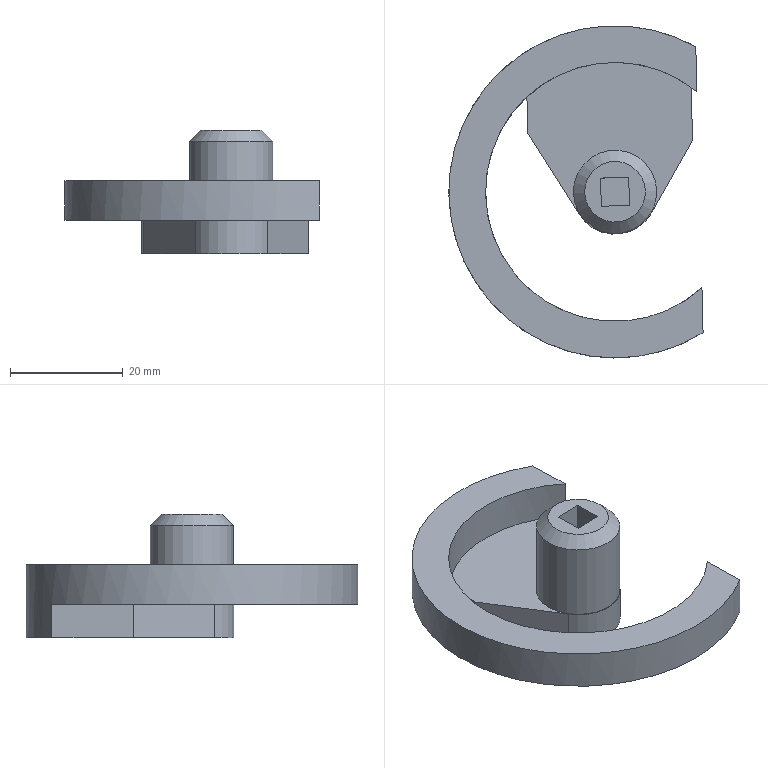Component | NX | LOCK_BODY | 1 solid | 22 faces | volume 12878 mm3 | plane 17 | cylinder 4 | cone 1 | commonest cylinder face diameters 46 x1 59 x1 15 x1 14.8 x1